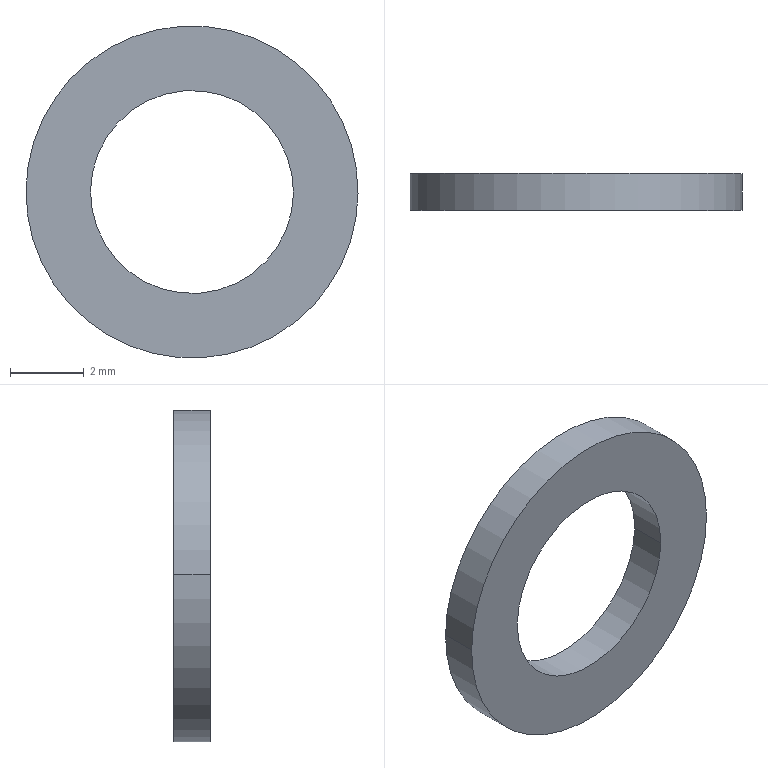Component | SolidWorks | M5CopperSealingGasket-2 | 1 solid | 6 faces | box 9 x 1 x 9 mm | volume 40 mm3 | cylinder 4 | plane 2 | commonest cylinder face diameters 5.5 x2 9 x2 | material CopperT3
build123d program:
from build123d import *

# Parameters (mm, degrees)
SKETCH1_R           = 4.5
SKETCH1_R_2         = 2.75
EXTRUDE_THIN1_DEPTH = 1


with BuildPart() as part:
    # Sketch1 → Extrude-Thin1 (new body)
    with BuildSketch(Plane.XY):
        Circle(SKETCH1_R)
        Circle(SKETCH1_R_2, mode=Mode.SUBTRACT)
    extrude(amount=EXTRUDE_THIN1_DEPTH)


solid = part.part

# Placed as in the assembly
solid = solid.moved(Location((-9, 66, 12), (90, 0, 0)))
STEP:
#1=COLOUR_RGB('',0.7922,0.8196,0.9333);
#2=FILL_AREA_STYLE_COLOUR('',#1);
#3=FILL_AREA_STYLE('',(#2));
#4=SURFACE_STYLE_FILL_AREA(#3);
#5=SURFACE_SIDE_STYLE('',(#4));
#6=SURFACE_STYLE_USAGE(.BOTH.,#5);
#7=PRESENTATION_STYLE_ASSIGNMENT((#6));
#8=CARTESIAN_POINT('',(-0.4626,2.598,0.4736));
#9=VERTEX_POINT('',#8);
#10=CARTESIAN_POINT('',(-0.2461,2.598,0.4713));
#11=VERTEX_POINT('',#10);
#12=CARTESIAN_POINT('',(-0.3543,2.598,0.4724));
#13=DIRECTION('',(0.,1.,-0.));
#14=DIRECTION('',(0.9999,0.,-0.01026));
#15=AXIS2_PLACEMENT_3D('',#12,#13,#14);
#16=CIRCLE('',#15,0.1083);
#17=EDGE_CURVE('',#9,#11,#16,.T.);
#18=ORIENTED_EDGE('',*,*,#17,.T.);
#19=CARTESIAN_POINT('',(-0.2461,2.559,0.4713));
#20=VERTEX_POINT('',#19);
#21=CARTESIAN_POINT('',(-0.2461,2.598,0.4713));
#22=DIRECTION('',(-0.,-1.,0.));
#23=VECTOR('',#22,39.37);
#24=LINE('',#21,#23);
#25=EDGE_CURVE('',#11,#20,#24,.T.);
#26=ORIENTED_EDGE('',*,*,#25,.T.);
#27=CARTESIAN_POINT('',(-0.4626,2.559,0.4736));
#28=VERTEX_POINT('',#27);
#29=CARTESIAN_POINT('',(-0.3543,2.559,0.4724));
#30=DIRECTION('',(0.,1.,-0.));
#31=DIRECTION('',(0.9999,0.,-0.01026));
#32=AXIS2_PLACEMENT_3D('',#29,#30,#31);
#33=CIRCLE('',#32,0.1083);
#34=EDGE_CURVE('',#28,#20,#33,.T.);
#35=ORIENTED_EDGE('',*,*,#34,.F.);
#36=CARTESIAN_POINT('',(-0.4626,2.598,0.4736));
#37=DIRECTION('',(-0.,-1.,0.));
#38=VECTOR('',#37,39.37);
#39=LINE('',#36,#38);
#40=EDGE_CURVE('',#9,#28,#39,.T.);
#41=ORIENTED_EDGE('',*,*,#40,.F.);
#42=EDGE_LOOP('',(#18,#26,#35,#41));
#43=FACE_OUTER_BOUND('',#42,.T.);
#44=CARTESIAN_POINT('',(-0.3543,2.598,0.4724));
#45=DIRECTION('',(-0.,-1.,0.));
#46=DIRECTION('',(-0.9999,0.,0.01026));
#47=AXIS2_PLACEMENT_3D('',#44,#45,#46);
#48=CYLINDRICAL_SURFACE('',#47,0.1083);
#49=ADVANCED_FACE('',(#43),#48,.F.);
#50=CARTESIAN_POINT('',(-0.1772,2.598,0.4706));
#51=VERTEX_POINT('',#50);
#52=CARTESIAN_POINT('',(-0.5315,2.598,0.4743));
#53=VERTEX_POINT('',#52);
#54=CARTESIAN_POINT('',(-0.3543,2.598,0.4724));
#55=DIRECTION('',(0.,1.,-0.));
#56=DIRECTION('',(0.9999,-0.,-0.01026));
#57=AXIS2_PLACEMENT_3D('',#54,#55,#56);
#58=CIRCLE('',#57,0.1772);
#59=EDGE_CURVE('',#51,#53,#58,.T.);
#60=ORIENTED_EDGE('',*,*,#59,.F.);
#61=CARTESIAN_POINT('',(-0.1772,2.559,0.4706));
#62=VERTEX_POINT('',#61);
#63=CARTESIAN_POINT('',(-0.1772,2.598,0.4706));
#64=DIRECTION('',(-0.,-1.,0.));
#65=VECTOR('',#64,39.37);
#66=LINE('',#63,#65);
#67=EDGE_CURVE('',#51,#62,#66,.T.);
#68=ORIENTED_EDGE('',*,*,#67,.T.);
#69=CARTESIAN_POINT('',(-0.5315,2.559,0.4743));
#70=VERTEX_POINT('',#69);
#71=CARTESIAN_POINT('',(-0.3543,2.559,0.4724));
#72=DIRECTION('',(0.,1.,-0.));
#73=DIRECTION('',(0.9999,-0.,-0.01026));
#74=AXIS2_PLACEMENT_3D('',#71,#72,#73);
#75=CIRCLE('',#74,0.1772);
#76=EDGE_CURVE('',#62,#70,#75,.T.);
#77=ORIENTED_EDGE('',*,*,#76,.T.);
#78=CARTESIAN_POINT('',(-0.5315,2.598,0.4743));
#79=DIRECTION('',(-0.,-1.,0.));
#80=VECTOR('',#79,39.37);
#81=LINE('',#78,#80);
#82=EDGE_CURVE('',#53,#70,#81,.T.);
#83=ORIENTED_EDGE('',*,*,#82,.F.);
#84=EDGE_LOOP('',(#60,#68,#77,#83));
#85=FACE_OUTER_BOUND('',#84,.T.);
#86=CARTESIAN_POINT('',(-0.3543,2.598,0.4724));
#87=DIRECTION('',(-0.,-1.,0.));
#88=DIRECTION('',(-0.9999,0.,0.01026));
#89=AXIS2_PLACEMENT_3D('',#86,#87,#88);
#90=CYLINDRICAL_SURFACE('',#89,0.1772);
#91=ADVANCED_FACE('',(#85),#90,.T.);
#92=CARTESIAN_POINT('',(-0.3543,2.598,0.4724));
#93=DIRECTION('',(0.,1.,-0.));
#94=DIRECTION('',(0.9999,-0.,-0.01026));
#95=AXIS2_PLACEMENT_3D('',#92,#93,#94);
#96=CIRCLE('',#95,0.1772);
#97=EDGE_CURVE('',#53,#51,#96,.T.);
#98=ORIENTED_EDGE('',*,*,#97,.T.);
#99=ORIENTED_EDGE('',*,*,#59,.T.);
#100=EDGE_LOOP('',(#98,#99));
#101=FACE_OUTER_BOUND('',#100,.T.);
#102=ORIENTED_EDGE('',*,*,#17,.F.);
#103=CARTESIAN_POINT('',(-0.3543,2.598,0.4724));
#104=DIRECTION('',(0.,1.,-0.));
#105=DIRECTION('',(0.9999,0.,-0.01026));
#106=AXIS2_PLACEMENT_3D('',#103,#104,#105);
#107=CIRCLE('',#106,0.1083);
#108=EDGE_CURVE('',#11,#9,#107,.T.);
#109=ORIENTED_EDGE('',*,*,#108,.F.);
#110=EDGE_LOOP('',(#102,#109));
#111=FACE_BOUND('',#110,.T.);
#112=CARTESIAN_POINT('',(-0.3543,2.598,0.4724));
#113=DIRECTION('',(0.,1.,-0.));
#114=DIRECTION('',(0.9999,-0.,-0.01026));
#115=AXIS2_PLACEMENT_3D('',#112,#113,#114);
#116=PLANE('',#115);
#117=ADVANCED_FACE('',(#101,#111),#116,.T.);
#118=CARTESIAN_POINT('',(-0.3543,2.559,0.4724));
#119=DIRECTION('',(0.,1.,-0.));
#120=DIRECTION('',(0.9999,-0.,-0.01026));
#121=AXIS2_PLACEMENT_3D('',#118,#119,#120);
#122=CIRCLE('',#121,0.1772);
#123=EDGE_CURVE('',#70,#62,#122,.T.);
#124=ORIENTED_EDGE('',*,*,#123,.F.);
#125=ORIENTED_EDGE('',*,*,#76,.F.);
#126=EDGE_LOOP('',(#124,#125));
#127=FACE_OUTER_BOUND('',#126,.T.);
#128=ORIENTED_EDGE('',*,*,#34,.T.);
#129=CARTESIAN_POINT('',(-0.3543,2.559,0.4724));
#130=DIRECTION('',(0.,1.,-0.));
#131=DIRECTION('',(0.9999,0.,-0.01026));
#132=AXIS2_PLACEMENT_3D('',#129,#130,#131);
#133=CIRCLE('',#132,0.1083);
#134=EDGE_CURVE('',#20,#28,#133,.T.);
#135=ORIENTED_EDGE('',*,*,#134,.T.);
#136=EDGE_LOOP('',(#128,#135));
#137=FACE_BOUND('',#136,.T.);
#138=CARTESIAN_POINT('',(-0.3543,2.559,0.4724));
#139=DIRECTION('',(0.,1.,-0.));
#140=DIRECTION('',(0.9999,-0.,-0.01026));
#141=AXIS2_PLACEMENT_3D('',#138,#139,#140);
#142=PLANE('',#141);
#143=ADVANCED_FACE('',(#127,#137),#142,.F.);
#144=ORIENTED_EDGE('',*,*,#67,.F.);
#145=ORIENTED_EDGE('',*,*,#97,.F.);
#146=ORIENTED_EDGE('',*,*,#82,.T.);
#147=ORIENTED_EDGE('',*,*,#123,.T.);
#148=EDGE_LOOP('',(#144,#145,#146,#147));
#149=FACE_OUTER_BOUND('',#148,.T.);
#150=CARTESIAN_POINT('',(-0.3543,2.598,0.4724));
#151=DIRECTION('',(-0.,-1.,0.));
#152=DIRECTION('',(-0.9999,0.,0.01026));
#153=AXIS2_PLACEMENT_3D('',#150,#151,#152);
#154=CYLINDRICAL_SURFACE('',#153,0.1772);
#155=ADVANCED_FACE('',(#149),#154,.T.);
#156=ORIENTED_EDGE('',*,*,#25,.F.);
#157=ORIENTED_EDGE('',*,*,#108,.T.);
#158=ORIENTED_EDGE('',*,*,#40,.T.);
#159=ORIENTED_EDGE('',*,*,#134,.F.);
#160=EDGE_LOOP('',(#156,#157,#158,#159));
#161=FACE_OUTER_BOUND('',#160,.T.);
#162=CARTESIAN_POINT('',(-0.3543,2.598,0.4724));
#163=DIRECTION('',(-0.,-1.,0.));
#164=DIRECTION('',(-0.9999,0.,0.01026));
#165=AXIS2_PLACEMENT_3D('',#162,#163,#164);
#166=CYLINDRICAL_SURFACE('',#165,0.1083);
#167=ADVANCED_FACE('',(#161),#166,.F.);
#168=CLOSED_SHELL('',(#49,#91,#117,#143,#155,#167));
#169=MANIFOLD_SOLID_BREP('',#168);
#170=STYLED_ITEM('',(#7),#169);
#171=(LENGTH_UNIT()NAMED_UNIT(*)SI_UNIT($,.METRE.));
#172=LENGTH_MEASURE_WITH_UNIT(LENGTH_MEASURE(0.0254),#171);
#173=DIMENSIONAL_EXPONENTS(1.,0.,0.,0.,0.,0.,0.);
#174=(CONVERSION_BASED_UNIT('',#172)LENGTH_UNIT()NAMED_UNIT(#173));
#175=UNCERTAINTY_MEASURE_WITH_UNIT(LENGTH_MEASURE(0.00001),#174,'','');
#176=(NAMED_UNIT(*)PLANE_ANGLE_UNIT()SI_UNIT($,.RADIAN.));
#177=(NAMED_UNIT(*)SI_UNIT($,.STERADIAN.)SOLID_ANGLE_UNIT());
#178=(GEOMETRIC_REPRESENTATION_CONTEXT(3)GLOBAL_UNCERTAINTY_ASSIGNED_CONTEXT((#175))GLOBAL_UNIT_ASSIGNED_CONTEXT((#174,#176,#177))REPRESENTATION_CONTEXT('',''));
#179=MECHANICAL_DESIGN_GEOMETRIC_PRESENTATION_REPRESENTATION('',(#170),#178);
#180=CARTESIAN_POINT('',(0.,0.,0.));
#181=DIRECTION('',(0.,0.,1.));
#182=DIRECTION('',(1.,0.,0.));
#183=AXIS2_PLACEMENT_3D('',#180,#181,#182);
#184=(LENGTH_UNIT()NAMED_UNIT(*)SI_UNIT($,.METRE.));
#185=LENGTH_MEASURE_WITH_UNIT(LENGTH_MEASURE(0.0254),#184);
#186=DIMENSIONAL_EXPONENTS(1.,0.,0.,0.,0.,0.,0.);
#187=(CONVERSION_BASED_UNIT('',#185)LENGTH_UNIT()NAMED_UNIT(#186));
#188=UNCERTAINTY_MEASURE_WITH_UNIT(LENGTH_MEASURE(0.00001),#187,'','');
#189=(NAMED_UNIT(*)PLANE_ANGLE_UNIT()SI_UNIT($,.RADIAN.));
#190=(NAMED_UNIT(*)SI_UNIT($,.STERADIAN.)SOLID_ANGLE_UNIT());
#191=(GEOMETRIC_REPRESENTATION_CONTEXT(3)GLOBAL_UNCERTAINTY_ASSIGNED_CONTEXT((#188))GLOBAL_UNIT_ASSIGNED_CONTEXT((#187,#189,#190))REPRESENTATION_CONTEXT('',''));
#192=ADVANCED_BREP_SHAPE_REPRESENTATION('',(#169,#183),#191);
#193=PRESENTATION_LAYER_ASSIGNMENT('','',(#170));